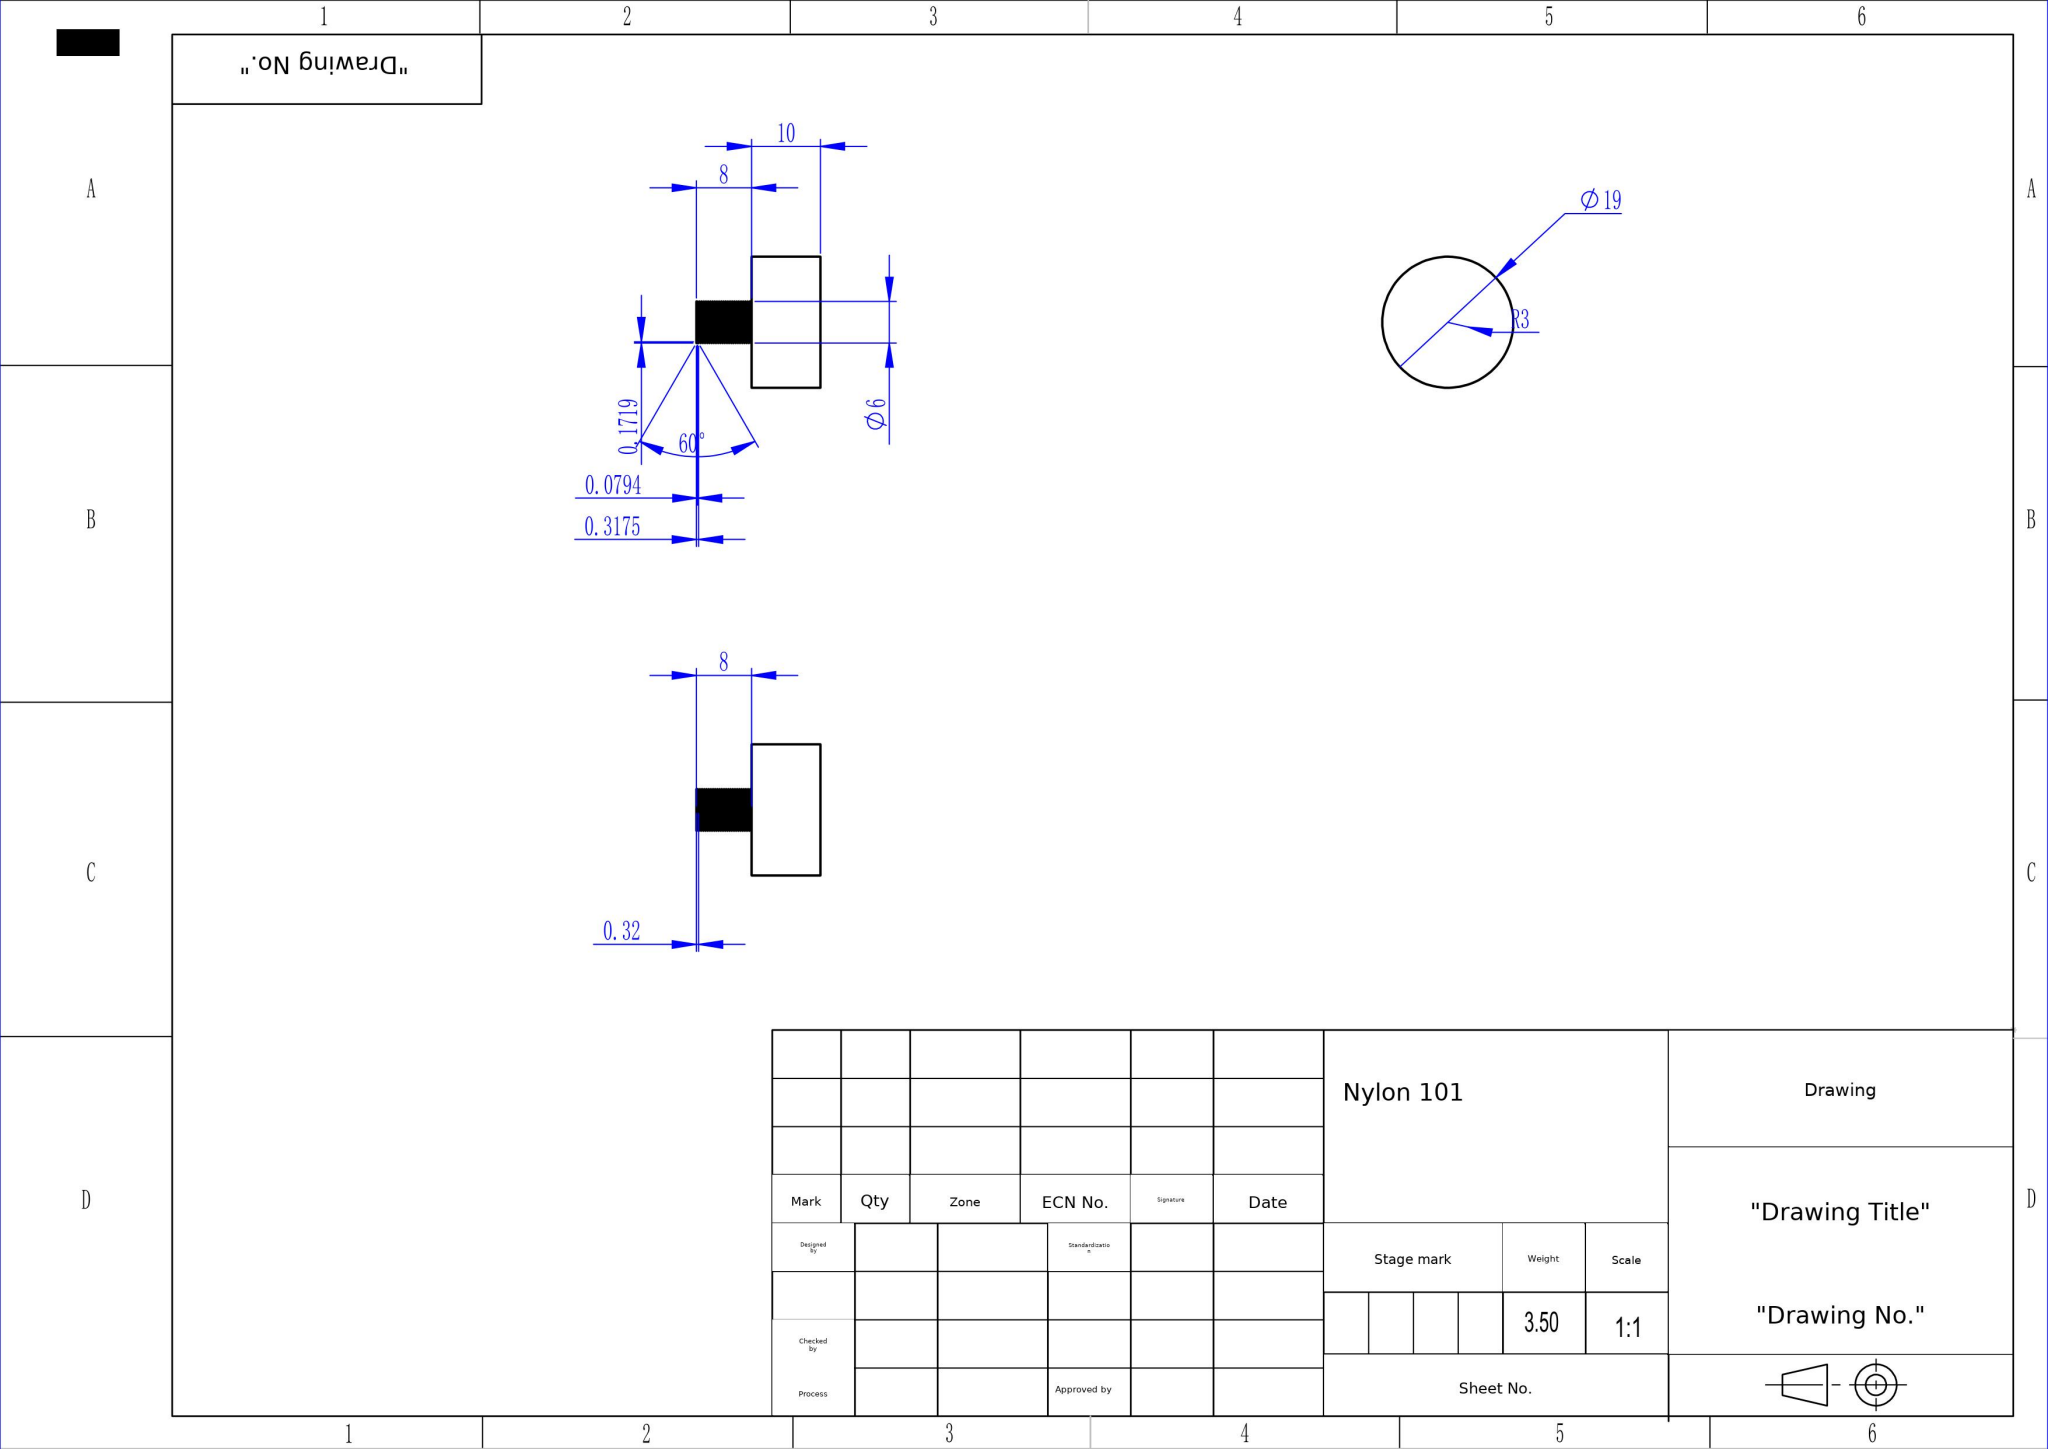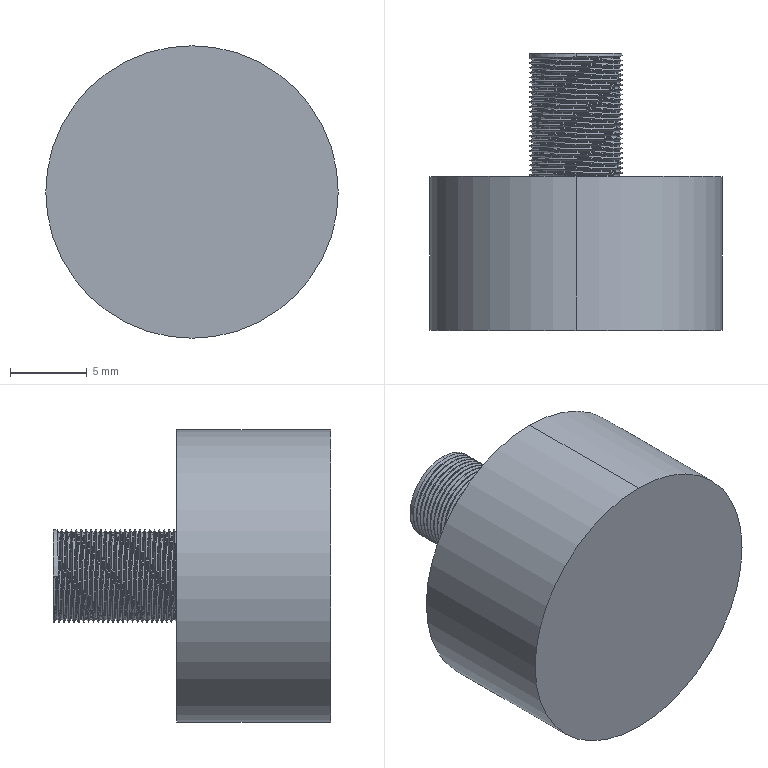Part | SolidWorks | mm | material Nylon 101 | 1 solid | 63 faces | box 19 x 18 x 19 mm | volume 3047 mm3 | cylinder 54 | plane 5 | spline 4 | commonest cylinder face diameters 6 x52 19 x2